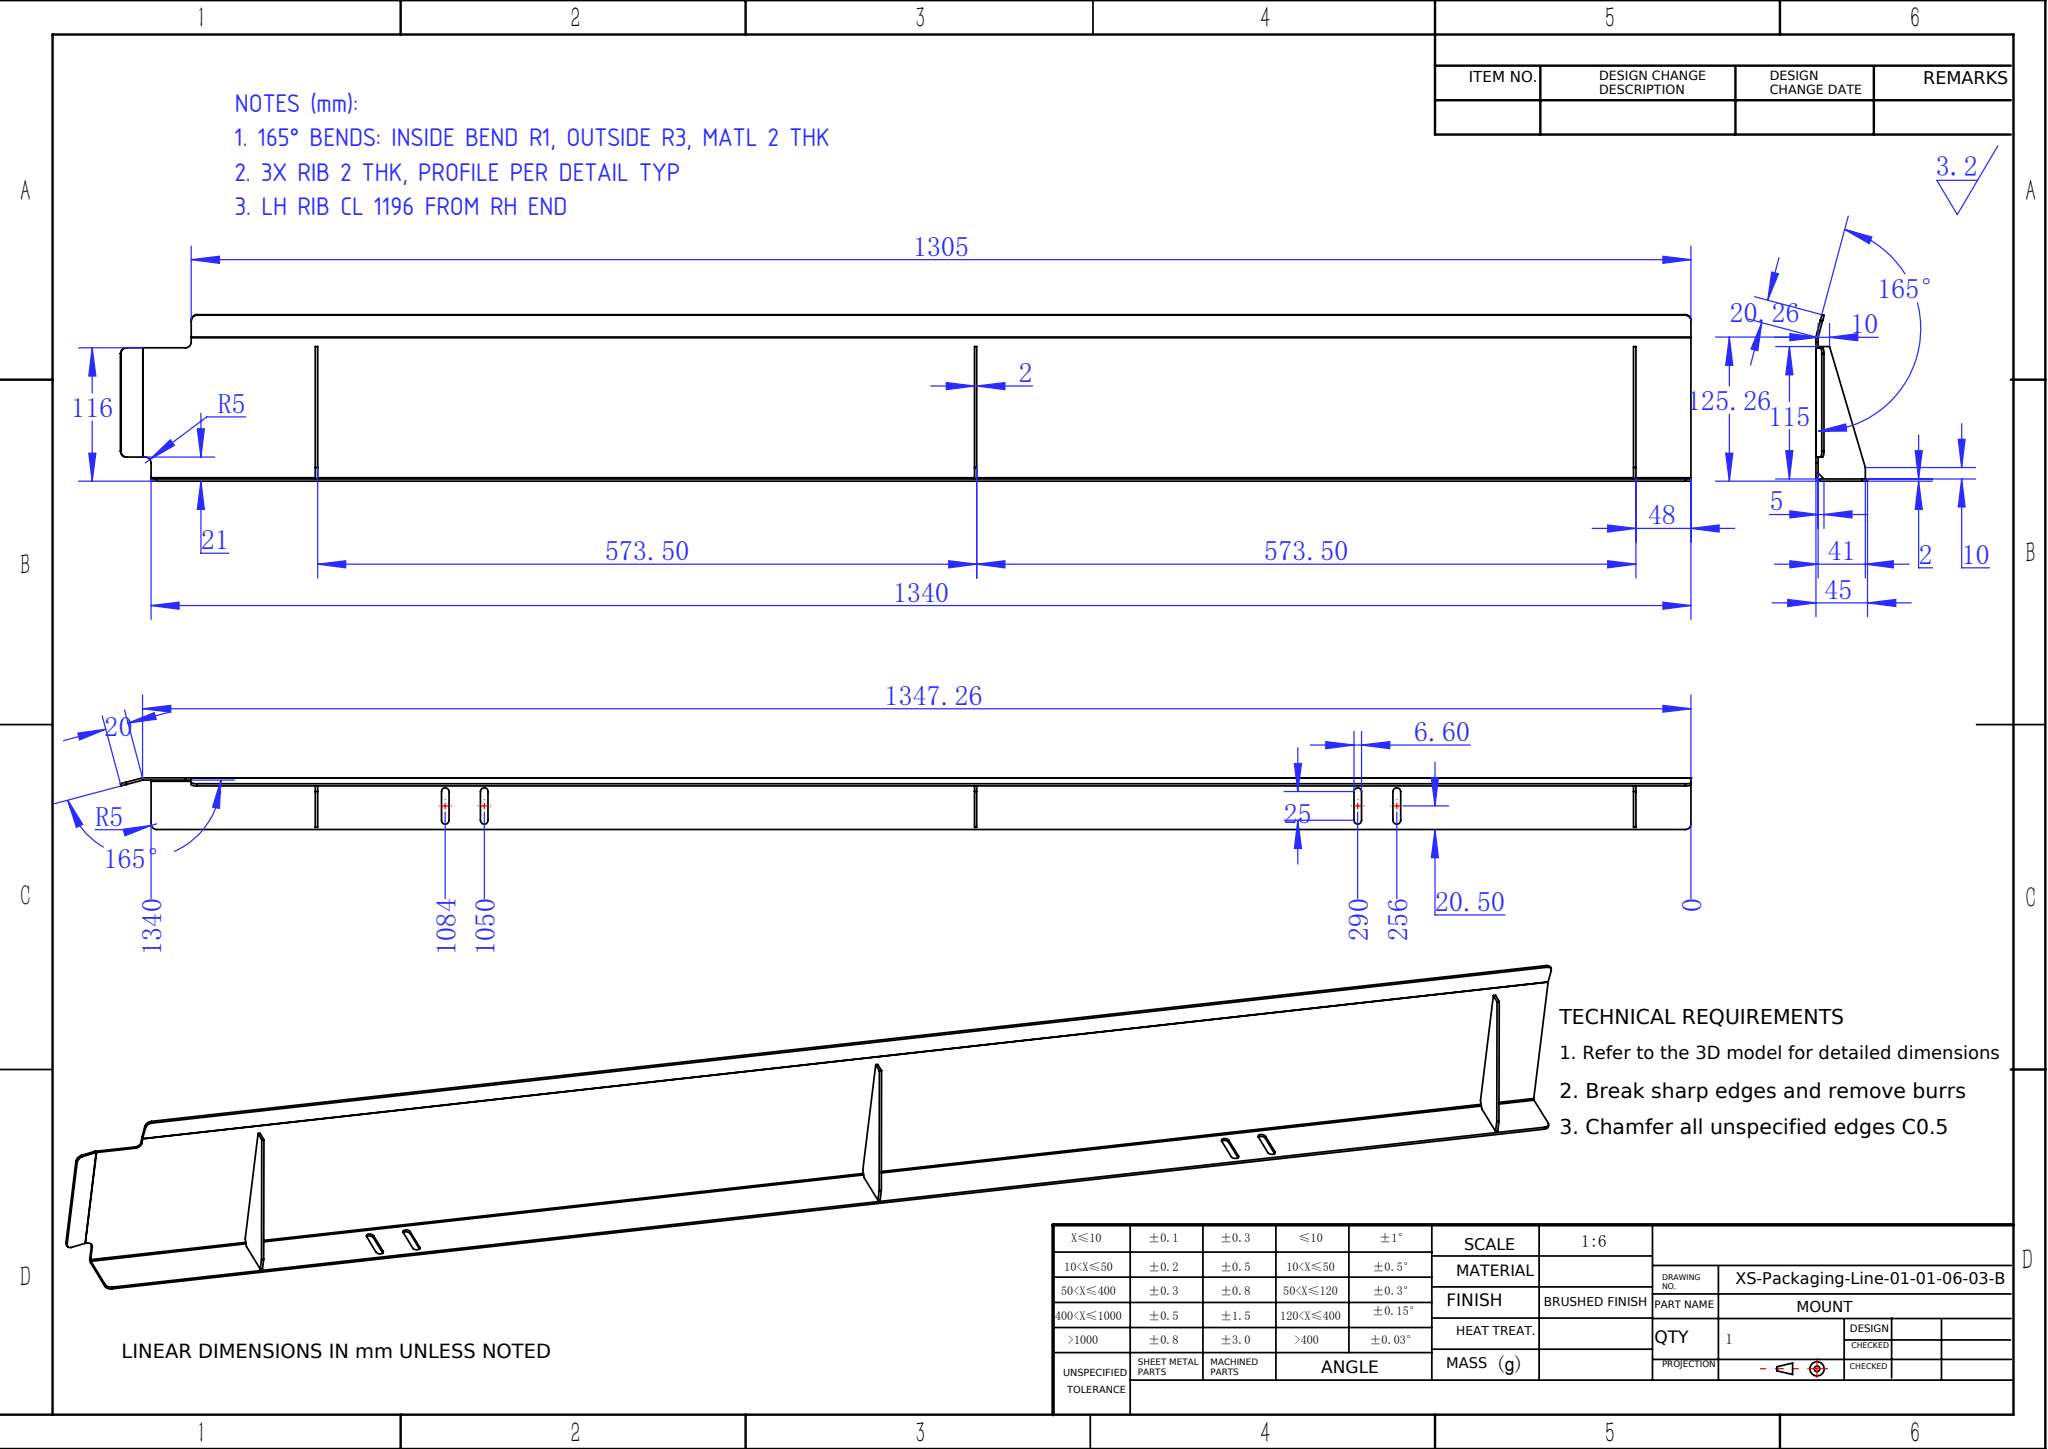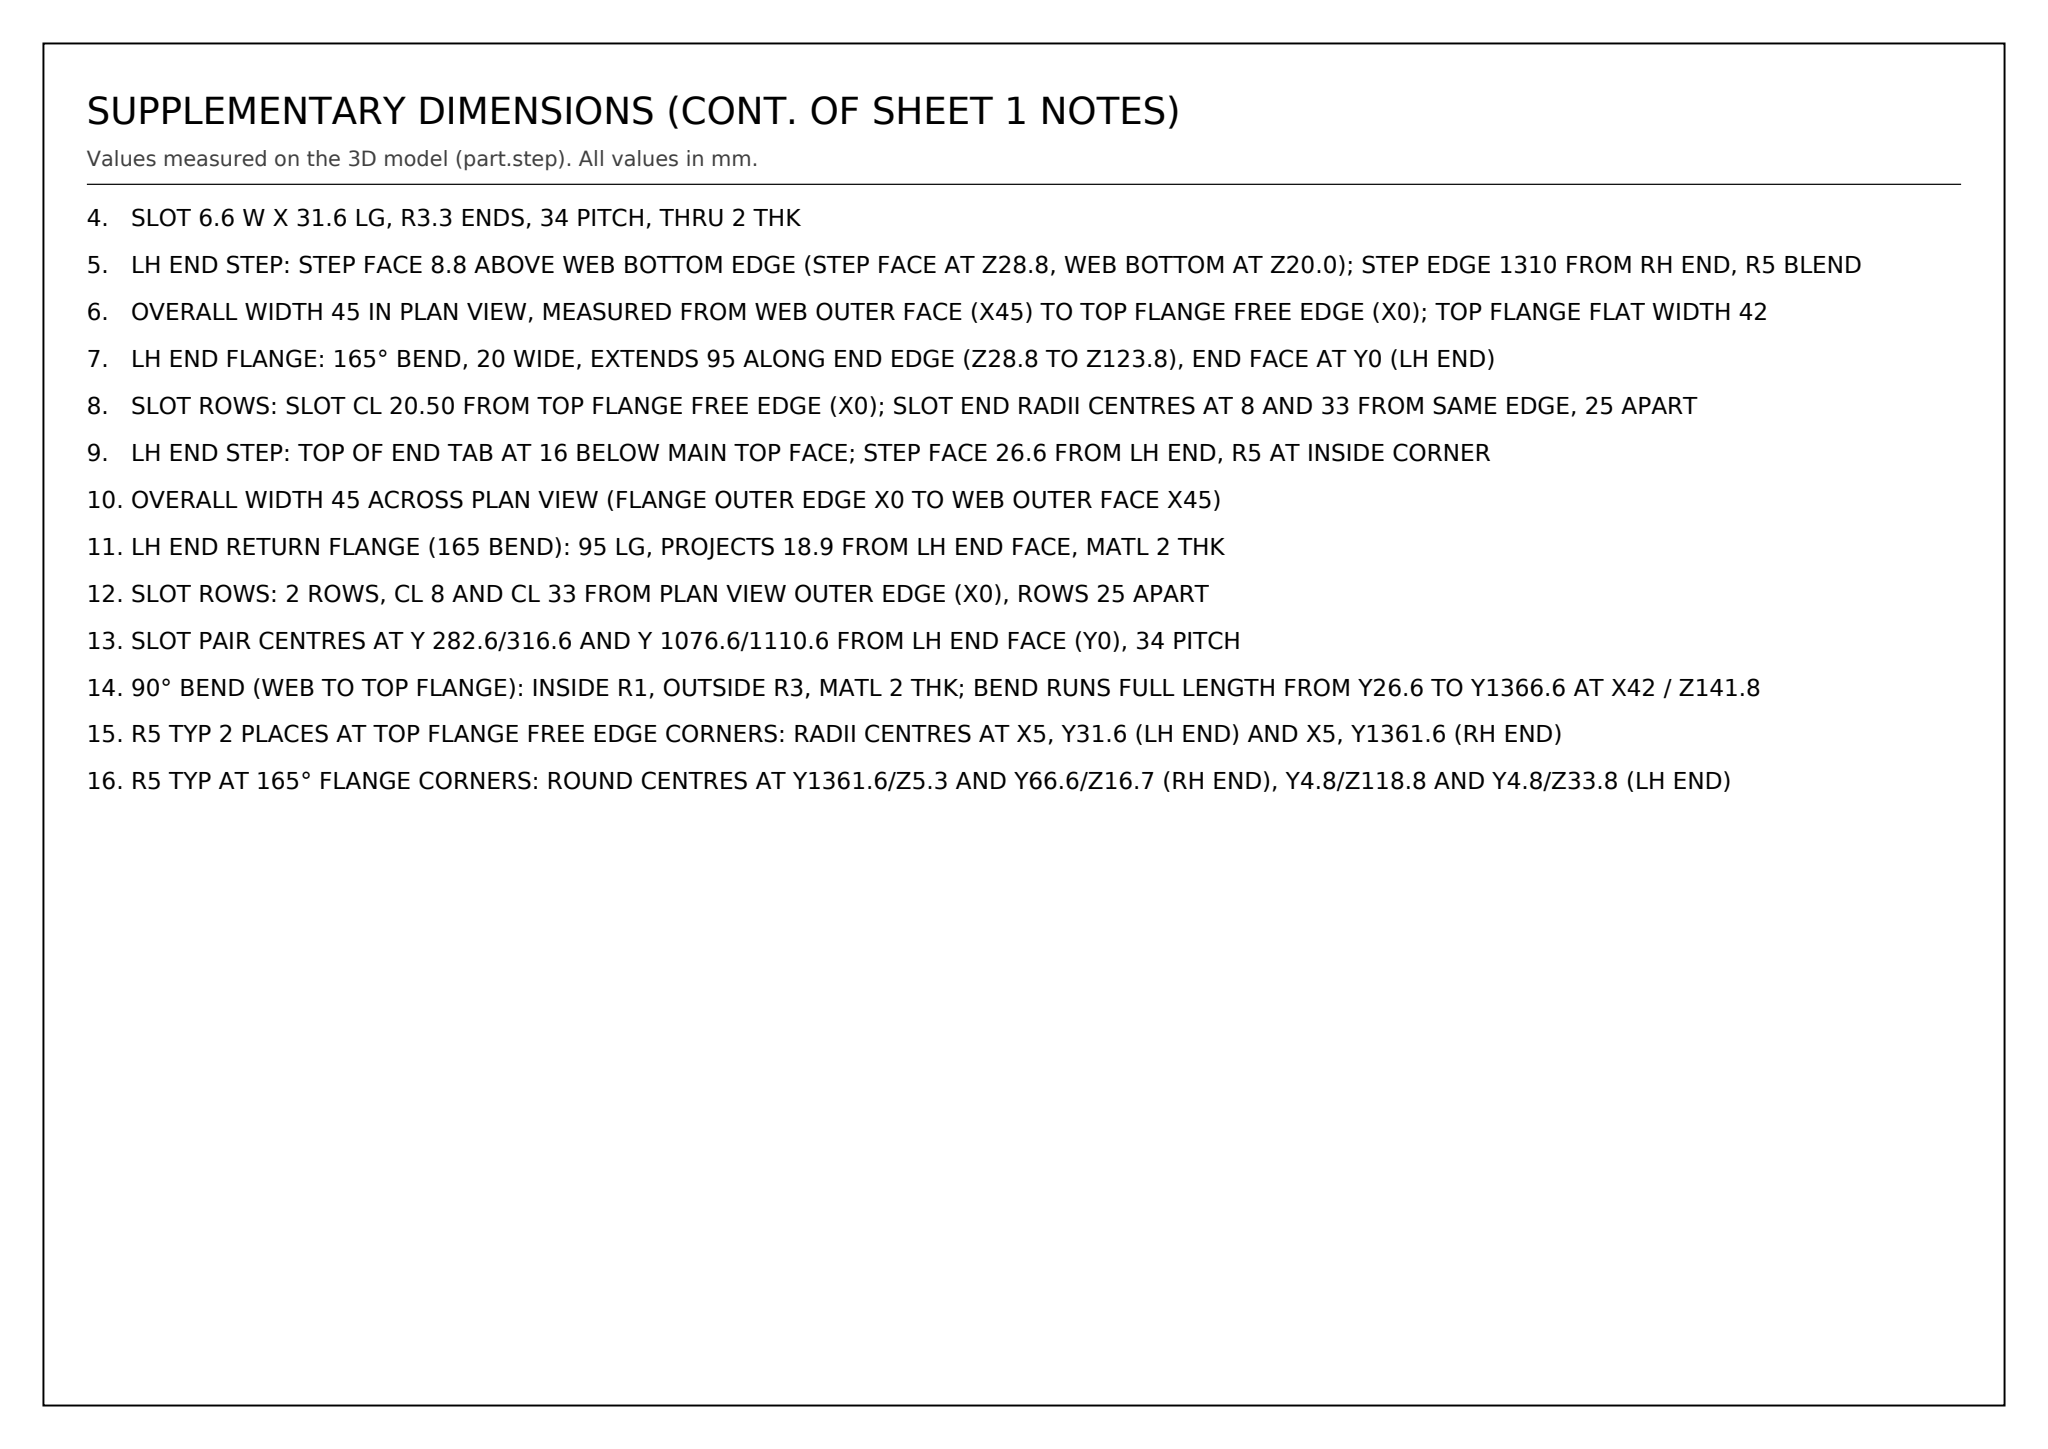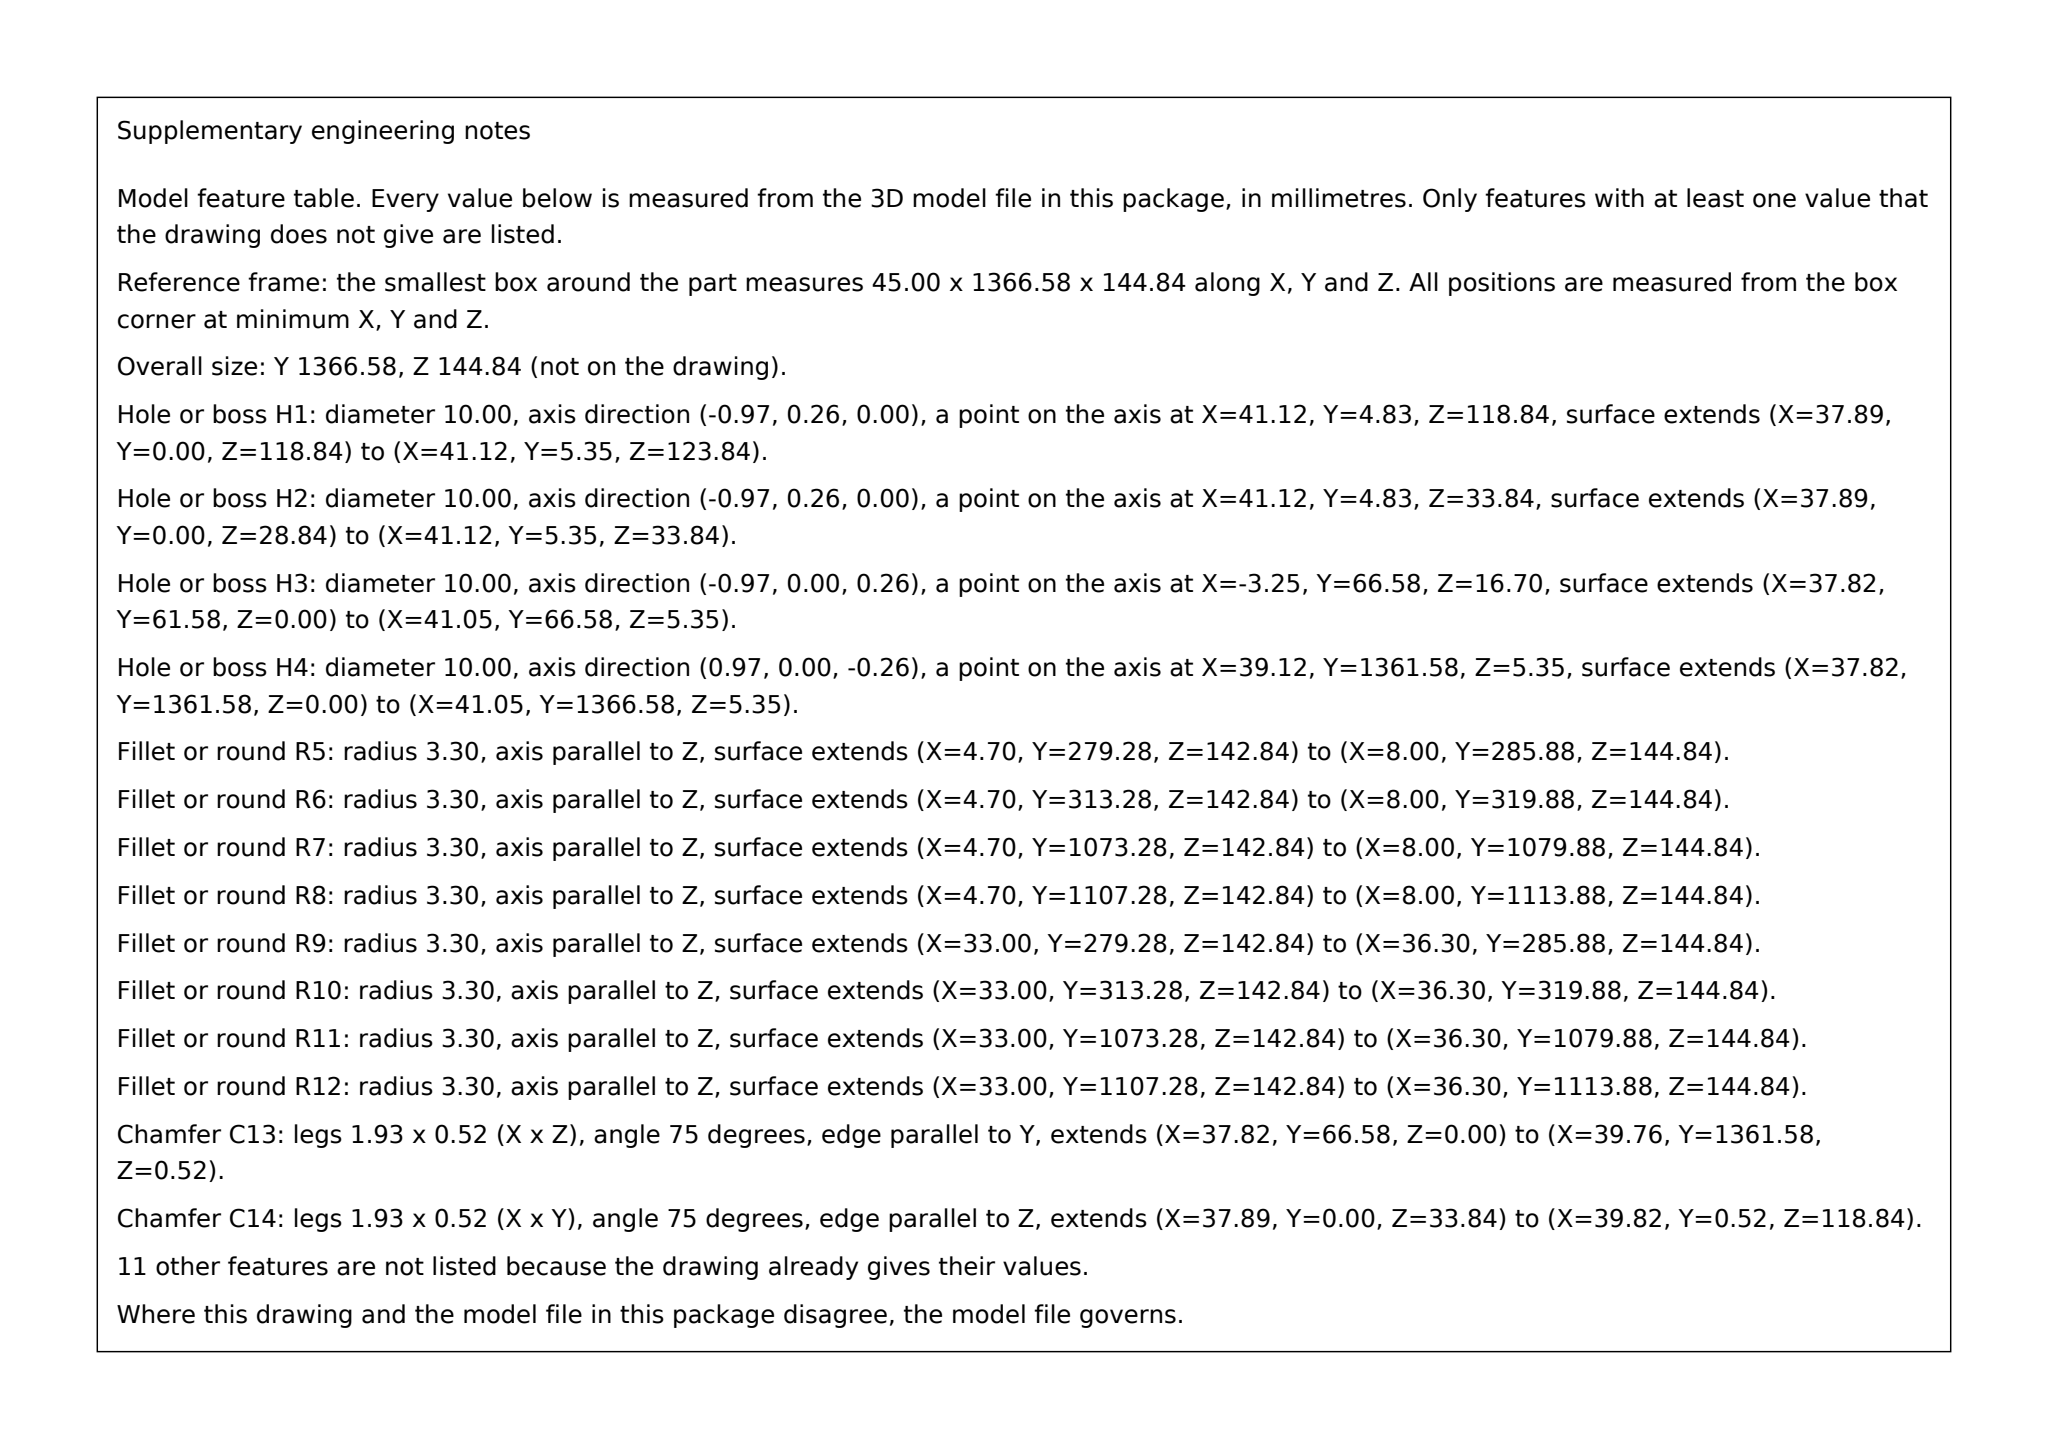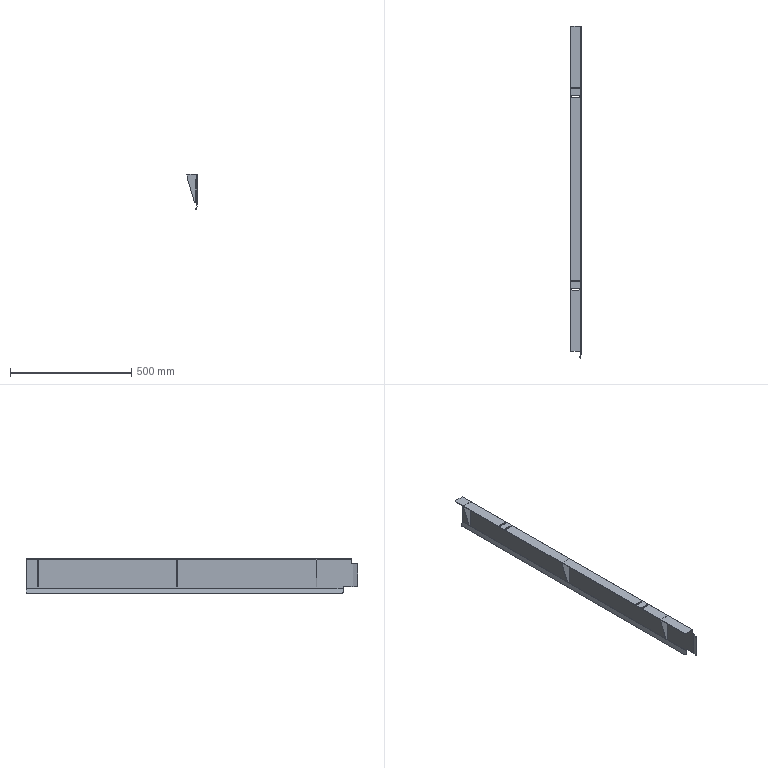Part | SolidWorks | mm | 1 solid | 78 faces | box 45 x 1366.58 x 144.84 mm | volume 522132 mm3 | plane 52 | cylinder 26 | commonest cylinder face diameters 6.6 x12 10 x8 2 x3 6 x3
Drawing notes:
165° BENDS: INSIDE BEND R1, OUTSIDE R3, MATL 2 THK | from the solid: Ø2.0 y-axis cyls at (x42,z19.97) L1305 & (x42,z141.84) L1340 = R1 inner; matching Ø6.0 cyls = R3 outer, t=2
3X RIB 2 THK, PROFILE PER DETAIL TYP | from the solid: Rib walls at y=169.58/171.58, 743.08/745.08, 1316.58/1318.58 (3 ribs, 2 thk); profile planes z=27.84/123.84, x=2.0/43.0
LH RIB CL 1196 FROM RH END | from the solid: LH rib c/l y=170.58; RH end y=1366.58 -> 1196.00
SLOT 6.6 W X 31.6 LG, R3.3 ENDS, 34 PITCH, THRU 2 THK | from the solid: Ø6.6 z-axis cyls len 2.0 at x=8.0 & 33.0 (25 c/c -> 31.6 lg, R3.3 ends); pairs at y=282.58/316.58 & 1076.58/1110.58 (34 apart)
LH END STEP: STEP FACE 8.8 ABOVE WEB BOTTOM EDGE (STEP FACE AT Z28.8, WEB BOTTOM AT Z20.0); STEP EDGE 1310 FROM RH END, R5 BLEND | from the solid: axis_planes z=28.8 extent x[43,45] y[19.7,56.6]; axis_planes x=43 and x=45 extent z[20.0,141.8]; concave arc dia 10 axis x at (y 56.6, z 23.8); bbox y 1366.582
OVERALL WIDTH 45 IN PLAN VIEW, MEASURED FROM WEB OUTER FACE (X45) TO TOP FLANGE FREE EDGE (X0); TOP FLANGE FLAT WIDTH 42 | from the solid: bbox_xyz x = 45.0; axis_planes x=45 and x=0; top flange planes z=142.8/144.8 extent x[0,42]
LH END FLANGE: 165° BEND, 20 WIDE, EXTENDS 95 ALONG END EDGE (Z28.8 TO Z123.8), END FACE AT Y0 (LH END) | from the solid: inclined_planes angle [15,75,90] bbox_from [37.9,0.5,28.8] size [5.1,18.9,95.0]; axis_plane z=28.8 extent x[43,45] y[19.7,56.6]; axis_plane z=123.8 extent x[43,45] y[19.7,21.6]
SLOT ROWS: SLOT CL 20.50 FROM TOP FLANGE FREE EDGE (X0); SLOT END RADII CENTRES AT 8 AND 33 FROM SAME EDGE, 25 APART | from the solid: slot arcs dia 6.6 axis z at x=8.0 and x=33.0 (y 282.6/316.6/1076.6/1110.6), from z142.8 to z144.8; slot side planes y=279.3/285.9 extent x[8,33]
LH END STEP: TOP OF END TAB AT 16 BELOW MAIN TOP FACE; STEP FACE 26.6 FROM LH END, R5 AT INSIDE CORNER | from the solid: axis_planes z=144.8 top face extent y[26.6,1366.6]; axis_plane y=26.6 (x 43-45) extent z[128.8,141.8]; concave arc dia 10 axis x at (y 21.6, z 128.8)
OVERALL WIDTH 45 ACROSS PLAN VIEW (FLANGE OUTER EDGE X0 TO WEB OUTER FACE X45) | from the solid: bbox_xyz x = 45.0; axis_planes x=0.0 and x=45.0
LH END RETURN FLANGE (165 BEND): 95 LG, PROJECTS 18.9 FROM LH END FACE, MATL 2 THK | from the solid: inclined_planes angle_to_xyz [15,75,90] bbox_from [37.9,0.5,28.8] size [5.1,18.9,95.0]
SLOT ROWS: 2 ROWS, CL 8 AND CL 33 FROM PLAN VIEW OUTER EDGE (X0), ROWS 25 APART | from the solid: 6.6 dia slot-end arcs axis z at x=8.0 and x=33.0; axis_plane x=0.0 outer flange edge
SLOT PAIR CENTRES AT Y 282.6/316.6 AND Y 1076.6/1110.6 FROM LH END FACE (Y0), 34 PITCH | from the solid: 6.6 dia arcs axis z at y 282.6, 316.6, 1076.6, 1110.6
90° BEND (WEB TO TOP FLANGE): INSIDE R1, OUTSIDE R3, MATL 2 THK; BEND RUNS FULL LENGTH FROM Y26.6 TO Y1366.6 AT X42 / Z141.8 | from the solid: cylinders: concave arc dia 2.0 axis y at [42.0,-,141.8] from Y26.6 to Y1366.6 arc 90° (inside R1) with convex arc dia 6.0 axis y at same position arc 90° (outside R3); plate faces Z142.8 and Z144.8 give 2 THK
R5 TYP 2 PLACES AT TOP FLANGE FREE EDGE CORNERS: RADII CENTRES AT X5, Y31.6 (LH END) AND X5, Y1361.6 (RH END) | from the solid: cylinders: convex arc dia 10.0 axis z at [5.0, 31.6] and [5.0, 1361.6], from Z142.8 to Z144.8, arc 90°
R5 TYP AT 165° FLANGE CORNERS: ROUND CENTRES AT Y1361.6/Z5.3 AND Y66.6/Z16.7 (RH END), Y4.8/Z118.8 AND Y4.8/Z33.8 (LH END) | from the solid: cylinders: convex arc dia 10.0 inclined axis at [-,1361.6,5.3], [-,66.6,16.7], [-,4.8,118.8], [-,4.8,33.8], arc 90°